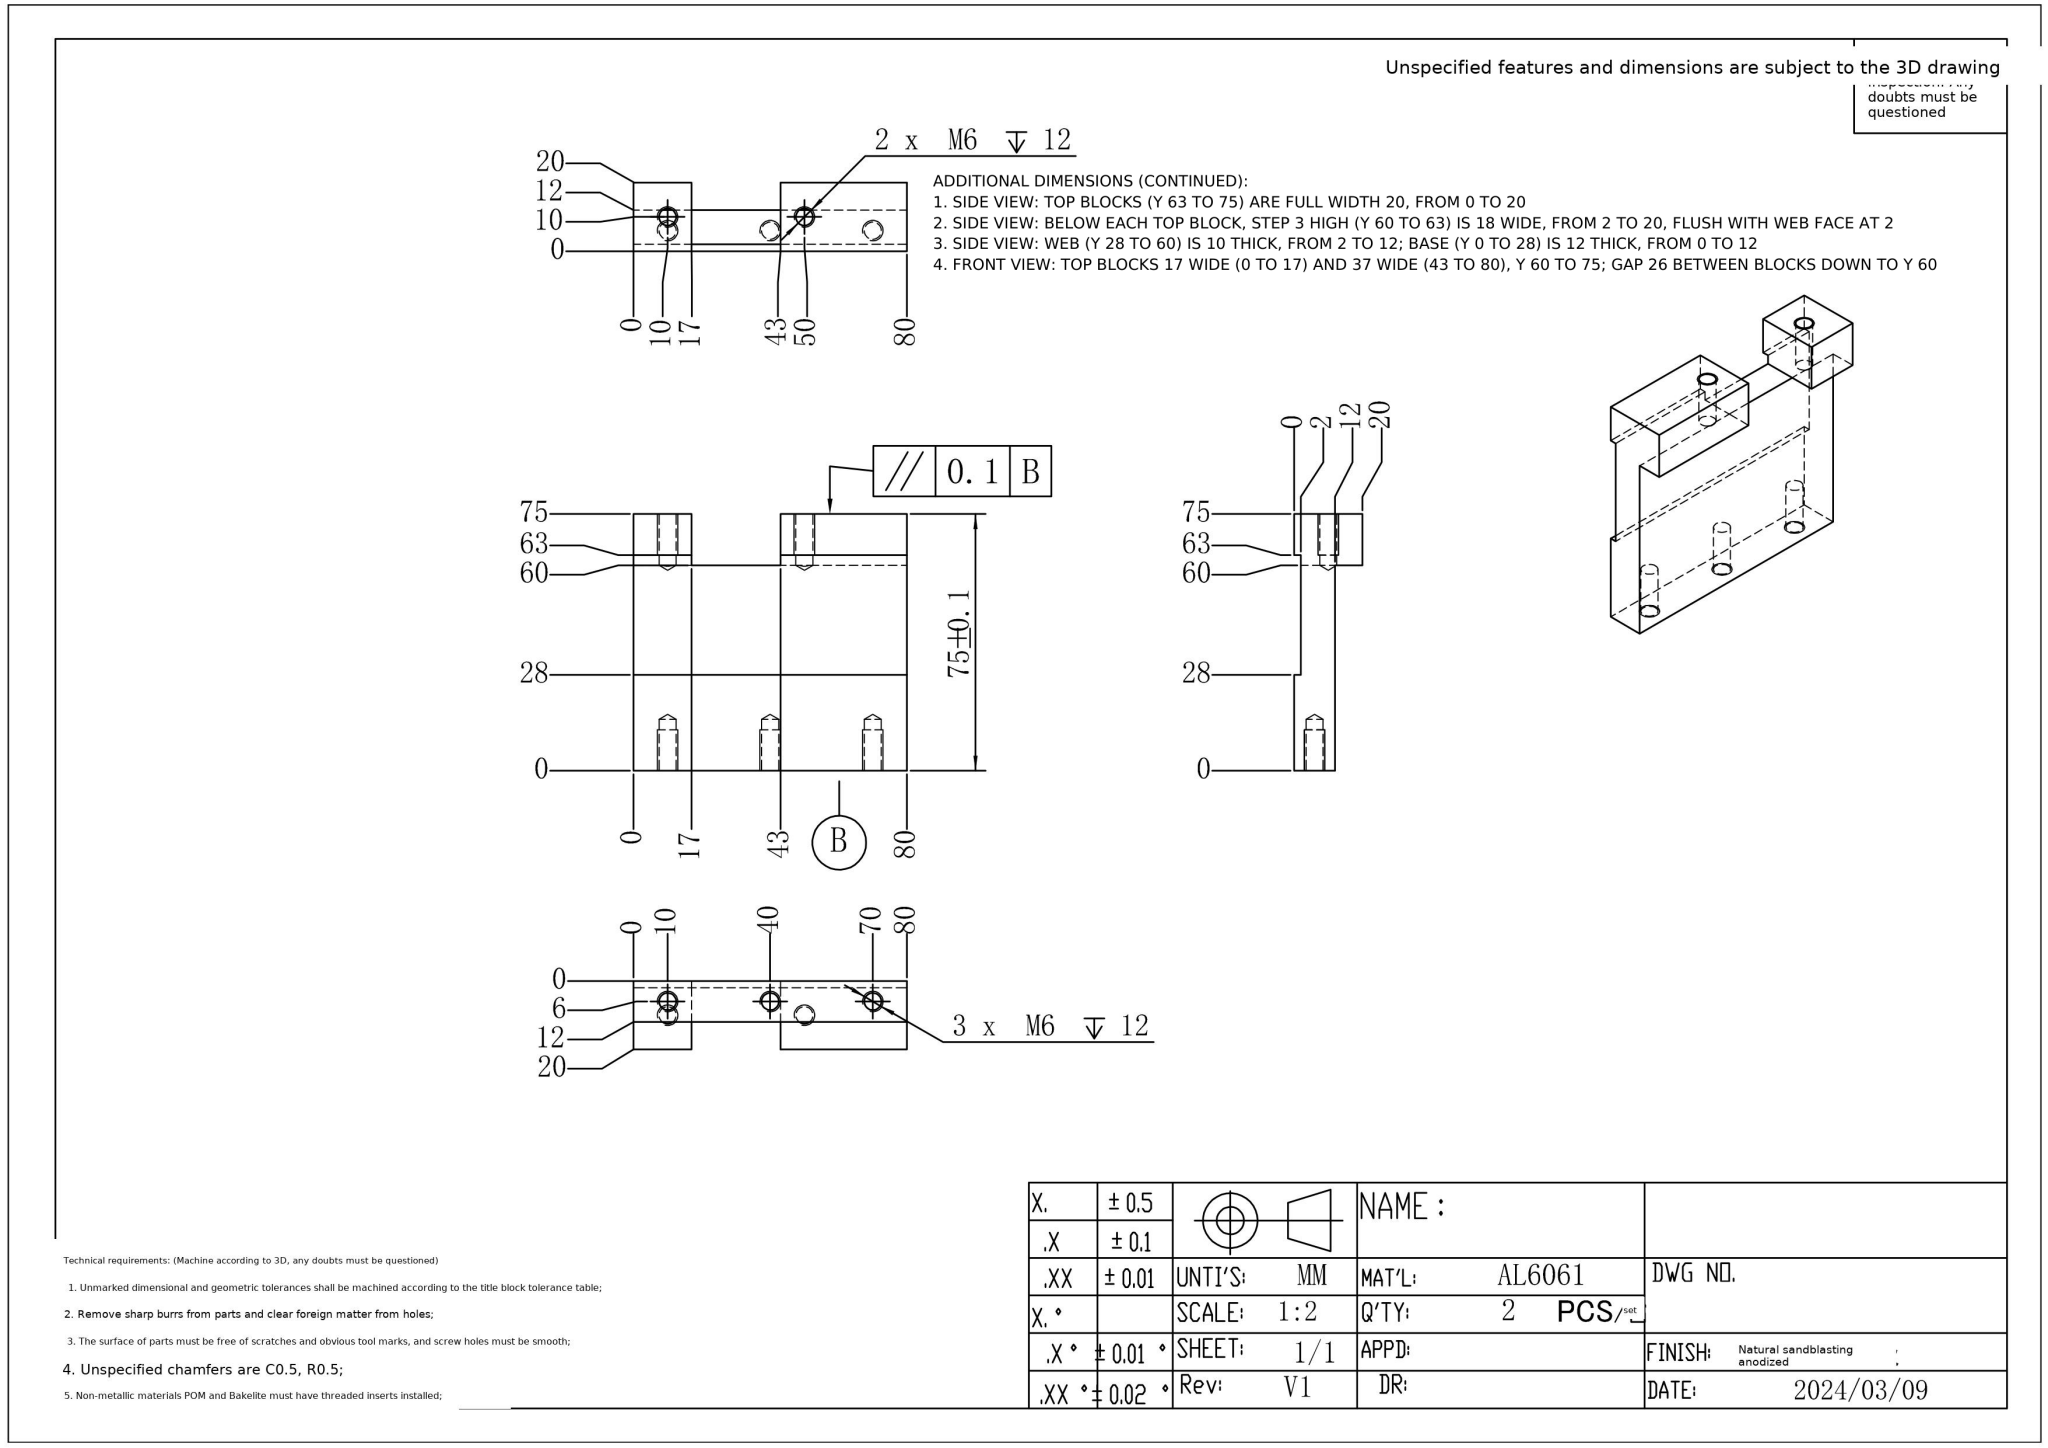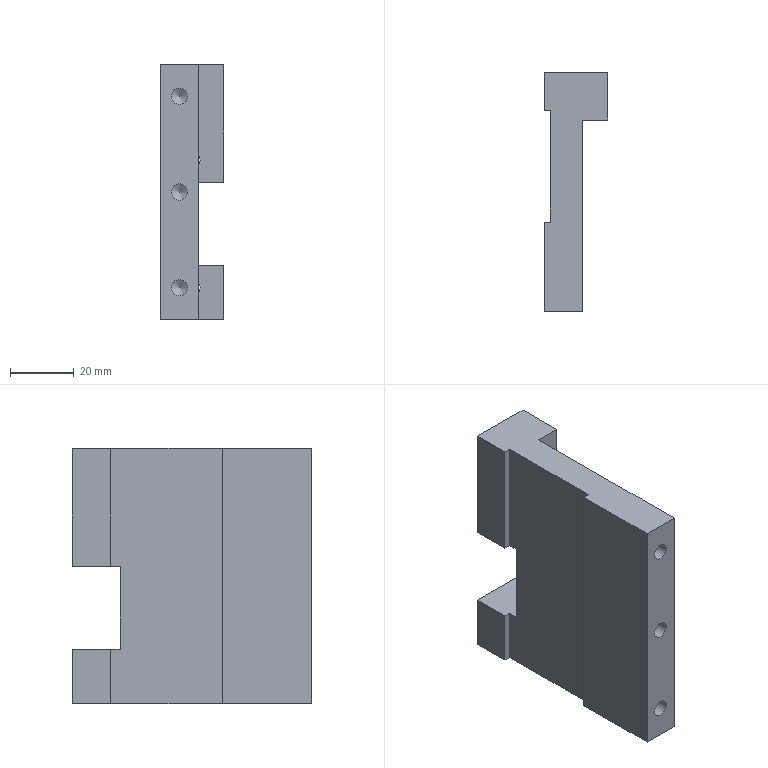Part | NX | mm | 1 solid | 30 faces | box 20 x 75 x 80 mm | volume 66772 mm3 | plane 20 | cone 5 | cylinder 5 | commonest cylinder face diameters 5.1 x5
STEP:
#1=CARTESIAN_POINT('',(0.,0.,0.));
#2=DIRECTION('',(0.,0.,1.));
#3=DIRECTION('',(1.,0.,0.));
#4=AXIS2_PLACEMENT_3D('',#1,#2,#3);
#5=(LENGTH_UNIT()NAMED_UNIT(*)SI_UNIT(.MILLI.,.METRE.));
#6=UNCERTAINTY_MEASURE_WITH_UNIT(LENGTH_MEASURE(0.0508),#5,'','');
#7=(NAMED_UNIT(*)PLANE_ANGLE_UNIT()SI_UNIT($,.RADIAN.));
#8=PLANE_ANGLE_MEASURE_WITH_UNIT(PLANE_ANGLE_MEASURE(0.01745),#7);
#9=DIMENSIONAL_EXPONENTS(0.,0.,0.,0.,0.,0.,0.);
#10=(CONVERSION_BASED_UNIT('',#8)NAMED_UNIT(#9)PLANE_ANGLE_UNIT());
#11=(NAMED_UNIT(*)SI_UNIT($,.STERADIAN.)SOLID_ANGLE_UNIT());
#12=(GEOMETRIC_REPRESENTATION_CONTEXT(3)GLOBAL_UNCERTAINTY_ASSIGNED_CONTEXT((#6))GLOBAL_UNIT_ASSIGNED_CONTEXT((#5,#10,#11))REPRESENTATION_CONTEXT('',''));
#13=SHAPE_REPRESENTATION('',(#4),#12);
#14=CARTESIAN_POINT('',(2.,60.,-63.));
#15=VERTEX_POINT('',#14);
#16=CARTESIAN_POINT('',(2.,60.,-37.));
#17=VERTEX_POINT('',#16);
#18=CARTESIAN_POINT('',(2.,60.,-80.));
#19=DIRECTION('',(0.,0.,1.));
#20=VECTOR('',#19,1.);
#21=LINE('',#18,#20);
#22=EDGE_CURVE('',#15,#17,#21,.T.);
#23=ORIENTED_EDGE('',*,*,#22,.T.);
#24=CARTESIAN_POINT('',(12.,60.,-37.));
#25=VERTEX_POINT('',#24);
#26=CARTESIAN_POINT('',(12.,60.,-37.));
#27=DIRECTION('',(-1.,0.,0.));
#28=VECTOR('',#27,1.);
#29=LINE('',#26,#28);
#30=EDGE_CURVE('',#25,#17,#29,.T.);
#31=ORIENTED_EDGE('',*,*,#30,.F.);
#32=CARTESIAN_POINT('',(12.,60.,-63.));
#33=VERTEX_POINT('',#32);
#34=CARTESIAN_POINT('',(12.,60.,-80.));
#35=DIRECTION('',(0.,0.,1.));
#36=VECTOR('',#35,1.);
#37=LINE('',#34,#36);
#38=EDGE_CURVE('',#33,#25,#37,.T.);
#39=ORIENTED_EDGE('',*,*,#38,.F.);
#40=CARTESIAN_POINT('',(2.,60.,-63.));
#41=DIRECTION('',(1.,0.,0.));
#42=VECTOR('',#41,1.);
#43=LINE('',#40,#42);
#44=EDGE_CURVE('',#15,#33,#43,.T.);
#45=ORIENTED_EDGE('',*,*,#44,.F.);
#46=EDGE_LOOP('',(#23,#31,#39,#45));
#47=FACE_OUTER_BOUND('',#46,.T.);
#48=CARTESIAN_POINT('',(12.,60.,-80.));
#49=DIRECTION('',(0.,1.,0.));
#50=DIRECTION('',(0.,0.,1.));
#51=AXIS2_PLACEMENT_3D('',#48,#49,#50);
#52=PLANE('',#51);
#53=ADVANCED_FACE('',(#47),#52,.T.);
#54=CARTESIAN_POINT('',(0.,28.,0.));
#55=VERTEX_POINT('',#54);
#56=CARTESIAN_POINT('',(0.,0.,0.));
#57=VERTEX_POINT('',#56);
#58=CARTESIAN_POINT('',(0.,28.,0.));
#59=DIRECTION('',(-0.,-1.,0.));
#60=VECTOR('',#59,1.);
#61=LINE('',#58,#60);
#62=EDGE_CURVE('',#55,#57,#61,.T.);
#63=ORIENTED_EDGE('',*,*,#62,.F.);
#64=CARTESIAN_POINT('',(0.,28.,-80.));
#65=VERTEX_POINT('',#64);
#66=CARTESIAN_POINT('',(0.,28.,-80.));
#67=DIRECTION('',(0.,0.,1.));
#68=VECTOR('',#67,1.);
#69=LINE('',#66,#68);
#70=EDGE_CURVE('',#65,#55,#69,.T.);
#71=ORIENTED_EDGE('',*,*,#70,.F.);
#72=CARTESIAN_POINT('',(0.,0.,-80.));
#73=VERTEX_POINT('',#72);
#74=CARTESIAN_POINT('',(0.,28.,-80.));
#75=DIRECTION('',(-0.,-1.,0.));
#76=VECTOR('',#75,1.);
#77=LINE('',#74,#76);
#78=EDGE_CURVE('',#65,#73,#77,.T.);
#79=ORIENTED_EDGE('',*,*,#78,.T.);
#80=CARTESIAN_POINT('',(0.,0.,-80.));
#81=DIRECTION('',(0.,0.,1.));
#82=VECTOR('',#81,1.);
#83=LINE('',#80,#82);
#84=EDGE_CURVE('',#73,#57,#83,.T.);
#85=ORIENTED_EDGE('',*,*,#84,.T.);
#86=EDGE_LOOP('',(#63,#71,#79,#85));
#87=FACE_OUTER_BOUND('',#86,.T.);
#88=CARTESIAN_POINT('',(0.,28.,-80.));
#89=DIRECTION('',(-1.,0.,0.));
#90=DIRECTION('',(-0.,-1.,0.));
#91=AXIS2_PLACEMENT_3D('',#88,#89,#90);
#92=PLANE('',#91);
#93=ADVANCED_FACE('',(#87),#92,.T.);
#94=CARTESIAN_POINT('',(3.45,0.,-40.));
#95=VERTEX_POINT('',#94);
#96=CARTESIAN_POINT('',(6.,0.,-40.));
#97=DIRECTION('',(0.,1.,0.));
#98=DIRECTION('',(-1.,0.,0.));
#99=AXIS2_PLACEMENT_3D('',#96,#97,#98);
#100=CIRCLE('',#99,2.55);
#101=EDGE_CURVE('',#95,#95,#100,.T.);
#102=ORIENTED_EDGE('',*,*,#101,.T.);
#103=EDGE_LOOP('',(#102));
#104=FACE_BOUND('',#103,.T.);
#105=CARTESIAN_POINT('',(3.45,0.,-10.));
#106=VERTEX_POINT('',#105);
#107=CARTESIAN_POINT('',(6.,0.,-10.));
#108=DIRECTION('',(0.,1.,0.));
#109=DIRECTION('',(-1.,0.,0.));
#110=AXIS2_PLACEMENT_3D('',#107,#108,#109);
#111=CIRCLE('',#110,2.55);
#112=EDGE_CURVE('',#106,#106,#111,.T.);
#113=ORIENTED_EDGE('',*,*,#112,.T.);
#114=EDGE_LOOP('',(#113));
#115=FACE_BOUND('',#114,.T.);
#116=CARTESIAN_POINT('',(3.45,0.,-70.));
#117=VERTEX_POINT('',#116);
#118=CARTESIAN_POINT('',(6.,0.,-70.));
#119=DIRECTION('',(0.,1.,0.));
#120=DIRECTION('',(-1.,0.,0.));
#121=AXIS2_PLACEMENT_3D('',#118,#119,#120);
#122=CIRCLE('',#121,2.55);
#123=EDGE_CURVE('',#117,#117,#122,.T.);
#124=ORIENTED_EDGE('',*,*,#123,.T.);
#125=EDGE_LOOP('',(#124));
#126=FACE_BOUND('',#125,.T.);
#127=CARTESIAN_POINT('',(12.,0.,0.));
#128=VERTEX_POINT('',#127);
#129=CARTESIAN_POINT('',(0.,0.,0.));
#130=DIRECTION('',(1.,-0.,0.));
#131=VECTOR('',#130,1.);
#132=LINE('',#129,#131);
#133=EDGE_CURVE('',#57,#128,#132,.T.);
#134=ORIENTED_EDGE('',*,*,#133,.F.);
#135=ORIENTED_EDGE('',*,*,#84,.F.);
#136=CARTESIAN_POINT('',(12.,0.,-80.));
#137=VERTEX_POINT('',#136);
#138=CARTESIAN_POINT('',(0.,0.,-80.));
#139=DIRECTION('',(1.,-0.,0.));
#140=VECTOR('',#139,1.);
#141=LINE('',#138,#140);
#142=EDGE_CURVE('',#73,#137,#141,.T.);
#143=ORIENTED_EDGE('',*,*,#142,.T.);
#144=CARTESIAN_POINT('',(12.,0.,-80.));
#145=DIRECTION('',(0.,0.,1.));
#146=VECTOR('',#145,1.);
#147=LINE('',#144,#146);
#148=EDGE_CURVE('',#137,#128,#147,.T.);
#149=ORIENTED_EDGE('',*,*,#148,.T.);
#150=EDGE_LOOP('',(#134,#135,#143,#149));
#151=FACE_BOUND('',#150,.T.);
#152=CARTESIAN_POINT('',(0.,0.,-80.));
#153=DIRECTION('',(-0.,-1.,0.));
#154=DIRECTION('',(1.,-0.,0.));
#155=AXIS2_PLACEMENT_3D('',#152,#153,#154);
#156=PLANE('',#155);
#157=ADVANCED_FACE('',(#104,#115,#126,#151),#156,.T.);
#158=CARTESIAN_POINT('',(12.,60.,-68.418));
#159=VERTEX_POINT('',#158);
#160=CARTESIAN_POINT('',(12.,60.,-71.582));
#161=VERTEX_POINT('',#160);
#162=CARTESIAN_POINT('',(12.,60.,-68.418));
#163=CARTESIAN_POINT('',(12.,59.81,-68.928));
#164=CARTESIAN_POINT('',(12.,59.669,-69.462));
#165=CARTESIAN_POINT('',(12.,59.67,-70.546));
#166=CARTESIAN_POINT('',(12.,59.811,-71.075));
#167=CARTESIAN_POINT('',(12.,60.,-71.582));
#168=B_SPLINE_CURVE_WITH_KNOTS('',3,(#162,#163,#164,#165,#166,#167),.UNSPECIFIED.,.F.,.F.,(4,2,4),(0.,0.5,1.),.UNSPECIFIED.);
#169=EDGE_CURVE('',#159,#161,#168,.T.);
#170=ORIENTED_EDGE('',*,*,#169,.F.);
#171=CARTESIAN_POINT('',(12.,60.,-80.));
#172=DIRECTION('',(0.,0.,1.));
#173=VECTOR('',#172,1.);
#174=LINE('',#171,#173);
#175=EDGE_CURVE('',#159,#33,#174,.T.);
#176=ORIENTED_EDGE('',*,*,#175,.T.);
#177=ORIENTED_EDGE('',*,*,#38,.T.);
#178=CARTESIAN_POINT('',(12.,60.,-31.582));
#179=VERTEX_POINT('',#178);
#180=CARTESIAN_POINT('',(12.,60.,-80.));
#181=DIRECTION('',(0.,0.,1.));
#182=VECTOR('',#181,1.);
#183=LINE('',#180,#182);
#184=EDGE_CURVE('',#25,#179,#183,.T.);
#185=ORIENTED_EDGE('',*,*,#184,.T.);
#186=CARTESIAN_POINT('',(12.,60.,-28.418));
#187=VERTEX_POINT('',#186);
#188=CARTESIAN_POINT('',(12.,60.,-28.418));
#189=CARTESIAN_POINT('',(12.,59.81,-28.928));
#190=CARTESIAN_POINT('',(12.,59.669,-29.462));
#191=CARTESIAN_POINT('',(12.,59.67,-30.546));
#192=CARTESIAN_POINT('',(12.,59.811,-31.075));
#193=CARTESIAN_POINT('',(12.,60.,-31.582));
#194=B_SPLINE_CURVE_WITH_KNOTS('',3,(#188,#189,#190,#191,#192,#193),.UNSPECIFIED.,.F.,.F.,(4,2,4),(0.,0.5,1.),.UNSPECIFIED.);
#195=EDGE_CURVE('',#187,#179,#194,.T.);
#196=ORIENTED_EDGE('',*,*,#195,.F.);
#197=CARTESIAN_POINT('',(12.,60.,0.));
#198=VERTEX_POINT('',#197);
#199=CARTESIAN_POINT('',(12.,60.,-80.));
#200=DIRECTION('',(0.,0.,1.));
#201=VECTOR('',#200,1.);
#202=LINE('',#199,#201);
#203=EDGE_CURVE('',#187,#198,#202,.T.);
#204=ORIENTED_EDGE('',*,*,#203,.T.);
#205=CARTESIAN_POINT('',(12.,0.,0.));
#206=DIRECTION('',(-0.,1.,0.));
#207=VECTOR('',#206,1.);
#208=LINE('',#205,#207);
#209=EDGE_CURVE('',#128,#198,#208,.T.);
#210=ORIENTED_EDGE('',*,*,#209,.F.);
#211=ORIENTED_EDGE('',*,*,#148,.F.);
#212=CARTESIAN_POINT('',(12.,60.,-80.));
#213=VERTEX_POINT('',#212);
#214=CARTESIAN_POINT('',(12.,0.,-80.));
#215=DIRECTION('',(-0.,1.,0.));
#216=VECTOR('',#215,1.);
#217=LINE('',#214,#216);
#218=EDGE_CURVE('',#137,#213,#217,.T.);
#219=ORIENTED_EDGE('',*,*,#218,.T.);
#220=CARTESIAN_POINT('',(12.,60.,-80.));
#221=DIRECTION('',(0.,0.,1.));
#222=VECTOR('',#221,1.);
#223=LINE('',#220,#222);
#224=EDGE_CURVE('',#213,#161,#223,.T.);
#225=ORIENTED_EDGE('',*,*,#224,.T.);
#226=EDGE_LOOP('',(#170,#176,#177,#185,#196,#204,#210,#211,#219,#225));
#227=FACE_OUTER_BOUND('',#226,.T.);
#228=CARTESIAN_POINT('',(12.,0.,-80.));
#229=DIRECTION('',(1.,0.,0.));
#230=DIRECTION('',(-0.,1.,0.));
#231=AXIS2_PLACEMENT_3D('',#228,#229,#230);
#232=PLANE('',#231);
#233=ADVANCED_FACE('',(#227),#232,.T.);
#234=CARTESIAN_POINT('',(2.,63.,0.));
#235=VERTEX_POINT('',#234);
#236=CARTESIAN_POINT('',(2.,28.,0.));
#237=VERTEX_POINT('',#236);
#238=CARTESIAN_POINT('',(2.,60.,0.));
#239=DIRECTION('',(0.,-1.,0.));
#240=VECTOR('',#239,1.);
#241=LINE('',#238,#240);
#242=EDGE_CURVE('',#235,#237,#241,.T.);
#243=ORIENTED_EDGE('',*,*,#242,.F.);
#244=CARTESIAN_POINT('',(2.,63.,-37.));
#245=VERTEX_POINT('',#244);
#246=CARTESIAN_POINT('',(2.,63.,0.));
#247=DIRECTION('',(0.,0.,-1.));
#248=VECTOR('',#247,1.);
#249=LINE('',#246,#248);
#250=EDGE_CURVE('',#235,#245,#249,.T.);
#251=ORIENTED_EDGE('',*,*,#250,.T.);
#252=CARTESIAN_POINT('',(2.,63.,-37.));
#253=DIRECTION('',(0.,1.,0.));
#254=VECTOR('',#253,1.);
#255=LINE('',#252,#254);
#256=EDGE_CURVE('',#17,#245,#255,.T.);
#257=ORIENTED_EDGE('',*,*,#256,.F.);
#258=ORIENTED_EDGE('',*,*,#22,.F.);
#259=CARTESIAN_POINT('',(2.,63.,-63.));
#260=VERTEX_POINT('',#259);
#261=CARTESIAN_POINT('',(2.,63.,-63.));
#262=DIRECTION('',(0.,-1.,0.));
#263=VECTOR('',#262,1.);
#264=LINE('',#261,#263);
#265=EDGE_CURVE('',#260,#15,#264,.T.);
#266=ORIENTED_EDGE('',*,*,#265,.F.);
#267=CARTESIAN_POINT('',(2.,63.,-80.));
#268=VERTEX_POINT('',#267);
#269=CARTESIAN_POINT('',(2.,63.,-80.));
#270=DIRECTION('',(0.,0.,1.));
#271=VECTOR('',#270,1.);
#272=LINE('',#269,#271);
#273=EDGE_CURVE('',#268,#260,#272,.T.);
#274=ORIENTED_EDGE('',*,*,#273,.F.);
#275=CARTESIAN_POINT('',(2.,28.,-80.));
#276=VERTEX_POINT('',#275);
#277=CARTESIAN_POINT('',(2.,60.,-80.));
#278=DIRECTION('',(0.,-1.,0.));
#279=VECTOR('',#278,1.);
#280=LINE('',#277,#279);
#281=EDGE_CURVE('',#268,#276,#280,.T.);
#282=ORIENTED_EDGE('',*,*,#281,.T.);
#283=CARTESIAN_POINT('',(2.,28.,-80.));
#284=DIRECTION('',(0.,0.,1.));
#285=VECTOR('',#284,1.);
#286=LINE('',#283,#285);
#287=EDGE_CURVE('',#276,#237,#286,.T.);
#288=ORIENTED_EDGE('',*,*,#287,.T.);
#289=EDGE_LOOP('',(#243,#251,#257,#258,#266,#274,#282,#288));
#290=FACE_OUTER_BOUND('',#289,.T.);
#291=CARTESIAN_POINT('',(2.,60.,-80.));
#292=DIRECTION('',(-1.,-0.,0.));
#293=DIRECTION('',(0.,-1.,0.));
#294=AXIS2_PLACEMENT_3D('',#291,#292,#293);
#295=PLANE('',#294);
#296=ADVANCED_FACE('',(#290),#295,.T.);
#297=CARTESIAN_POINT('',(2.,28.,0.));
#298=DIRECTION('',(-1.,0.,0.));
#299=VECTOR('',#298,1.);
#300=LINE('',#297,#299);
#301=EDGE_CURVE('',#237,#55,#300,.T.);
#302=ORIENTED_EDGE('',*,*,#301,.F.);
#303=ORIENTED_EDGE('',*,*,#287,.F.);
#304=CARTESIAN_POINT('',(2.,28.,-80.));
#305=DIRECTION('',(-1.,0.,0.));
#306=VECTOR('',#305,1.);
#307=LINE('',#304,#306);
#308=EDGE_CURVE('',#276,#65,#307,.T.);
#309=ORIENTED_EDGE('',*,*,#308,.T.);
#310=ORIENTED_EDGE('',*,*,#70,.T.);
#311=EDGE_LOOP('',(#302,#303,#309,#310));
#312=FACE_OUTER_BOUND('',#311,.T.);
#313=CARTESIAN_POINT('',(2.,28.,-80.));
#314=DIRECTION('',(0.,1.,0.));
#315=DIRECTION('',(0.,0.,1.));
#316=AXIS2_PLACEMENT_3D('',#313,#314,#315);
#317=PLANE('',#316);
#318=ADVANCED_FACE('',(#312),#317,.T.);
#319=ORIENTED_EDGE('',*,*,#78,.F.);
#320=ORIENTED_EDGE('',*,*,#308,.F.);
#321=ORIENTED_EDGE('',*,*,#281,.F.);
#322=CARTESIAN_POINT('',(-0.,63.,-80.));
#323=VERTEX_POINT('',#322);
#324=CARTESIAN_POINT('',(-0.,63.,-80.));
#325=DIRECTION('',(1.,0.,0.));
#326=VECTOR('',#325,1.);
#327=LINE('',#324,#326);
#328=EDGE_CURVE('',#323,#268,#327,.T.);
#329=ORIENTED_EDGE('',*,*,#328,.F.);
#330=CARTESIAN_POINT('',(-0.,75.,-80.));
#331=VERTEX_POINT('',#330);
#332=CARTESIAN_POINT('',(-0.,75.,-80.));
#333=DIRECTION('',(0.,-1.,0.));
#334=VECTOR('',#333,1.);
#335=LINE('',#332,#334);
#336=EDGE_CURVE('',#331,#323,#335,.T.);
#337=ORIENTED_EDGE('',*,*,#336,.F.);
#338=CARTESIAN_POINT('',(20.,75.,-80.));
#339=VERTEX_POINT('',#338);
#340=CARTESIAN_POINT('',(20.,75.,-80.));
#341=DIRECTION('',(-1.,0.,0.));
#342=VECTOR('',#341,1.);
#343=LINE('',#340,#342);
#344=EDGE_CURVE('',#339,#331,#343,.T.);
#345=ORIENTED_EDGE('',*,*,#344,.F.);
#346=CARTESIAN_POINT('',(20.,60.,-80.));
#347=VERTEX_POINT('',#346);
#348=CARTESIAN_POINT('',(20.,60.,-80.));
#349=DIRECTION('',(0.,1.,0.));
#350=VECTOR('',#349,1.);
#351=LINE('',#348,#350);
#352=EDGE_CURVE('',#347,#339,#351,.T.);
#353=ORIENTED_EDGE('',*,*,#352,.F.);
#354=CARTESIAN_POINT('',(2.,60.,-80.));
#355=DIRECTION('',(1.,0.,0.));
#356=VECTOR('',#355,1.);
#357=LINE('',#354,#356);
#358=EDGE_CURVE('',#213,#347,#357,.T.);
#359=ORIENTED_EDGE('',*,*,#358,.F.);
#360=ORIENTED_EDGE('',*,*,#218,.F.);
#361=ORIENTED_EDGE('',*,*,#142,.F.);
#362=EDGE_LOOP('',(#319,#320,#321,#329,#337,#345,#353,#359,#360,#361));
#363=FACE_OUTER_BOUND('',#362,.T.);
#364=CARTESIAN_POINT('',(0.,0.,-80.));
#365=DIRECTION('',(0.,0.,1.));
#366=DIRECTION('',(1.,0.,0.));
#367=AXIS2_PLACEMENT_3D('',#364,#365,#366);
#368=PLANE('',#367);
#369=ADVANCED_FACE('',(#363),#368,.F.);
#370=ORIENTED_EDGE('',*,*,#62,.T.);
#371=ORIENTED_EDGE('',*,*,#133,.T.);
#372=ORIENTED_EDGE('',*,*,#209,.T.);
#373=CARTESIAN_POINT('',(20.,60.,0.));
#374=VERTEX_POINT('',#373);
#375=CARTESIAN_POINT('',(2.,60.,0.));
#376=DIRECTION('',(1.,0.,0.));
#377=VECTOR('',#376,1.);
#378=LINE('',#375,#377);
#379=EDGE_CURVE('',#198,#374,#378,.T.);
#380=ORIENTED_EDGE('',*,*,#379,.T.);
#381=CARTESIAN_POINT('',(20.,75.,0.));
#382=VERTEX_POINT('',#381);
#383=CARTESIAN_POINT('',(20.,60.,0.));
#384=DIRECTION('',(0.,1.,0.));
#385=VECTOR('',#384,1.);
#386=LINE('',#383,#385);
#387=EDGE_CURVE('',#374,#382,#386,.T.);
#388=ORIENTED_EDGE('',*,*,#387,.T.);
#389=CARTESIAN_POINT('',(-0.,75.,0.));
#390=VERTEX_POINT('',#389);
#391=CARTESIAN_POINT('',(20.,75.,0.));
#392=DIRECTION('',(-1.,0.,0.));
#393=VECTOR('',#392,1.);
#394=LINE('',#391,#393);
#395=EDGE_CURVE('',#382,#390,#394,.T.);
#396=ORIENTED_EDGE('',*,*,#395,.T.);
#397=CARTESIAN_POINT('',(-0.,63.,0.));
#398=VERTEX_POINT('',#397);
#399=CARTESIAN_POINT('',(-0.,75.,0.));
#400=DIRECTION('',(0.,-1.,0.));
#401=VECTOR('',#400,1.);
#402=LINE('',#399,#401);
#403=EDGE_CURVE('',#390,#398,#402,.T.);
#404=ORIENTED_EDGE('',*,*,#403,.T.);
#405=CARTESIAN_POINT('',(-0.,63.,0.));
#406=DIRECTION('',(1.,0.,0.));
#407=VECTOR('',#406,1.);
#408=LINE('',#405,#407);
#409=EDGE_CURVE('',#398,#235,#408,.T.);
#410=ORIENTED_EDGE('',*,*,#409,.T.);
#411=ORIENTED_EDGE('',*,*,#242,.T.);
#412=ORIENTED_EDGE('',*,*,#301,.T.);
#413=EDGE_LOOP('',(#370,#371,#372,#380,#388,#396,#404,#410,#411,#412));
#414=FACE_OUTER_BOUND('',#413,.T.);
#415=CARTESIAN_POINT('',(0.,0.,0.));
#416=DIRECTION('',(0.,0.,1.));
#417=DIRECTION('',(1.,0.,0.));
#418=AXIS2_PLACEMENT_3D('',#415,#416,#417);
#419=PLANE('',#418);
#420=ADVANCED_FACE('',(#414),#419,.T.);
#421=CARTESIAN_POINT('',(10.,60.,-70.));
#422=DIRECTION('',(0.,-1.,0.));
#423=DIRECTION('',(0.,0.,-1.));
#424=AXIS2_PLACEMENT_3D('',#421,#422,#423);
#425=CIRCLE('',#424,2.55);
#426=EDGE_CURVE('',#161,#159,#425,.T.);
#427=ORIENTED_EDGE('',*,*,#426,.F.);
#428=ORIENTED_EDGE('',*,*,#224,.F.);
#429=ORIENTED_EDGE('',*,*,#358,.T.);
#430=CARTESIAN_POINT('',(20.,60.,-63.));
#431=VERTEX_POINT('',#430);
#432=CARTESIAN_POINT('',(20.,60.,-80.));
#433=DIRECTION('',(0.,0.,1.));
#434=VECTOR('',#433,1.);
#435=LINE('',#432,#434);
#436=EDGE_CURVE('',#347,#431,#435,.T.);
#437=ORIENTED_EDGE('',*,*,#436,.T.);
#438=CARTESIAN_POINT('',(2.,60.,-63.));
#439=DIRECTION('',(1.,0.,0.));
#440=VECTOR('',#439,1.);
#441=LINE('',#438,#440);
#442=EDGE_CURVE('',#33,#431,#441,.T.);
#443=ORIENTED_EDGE('',*,*,#442,.F.);
#444=ORIENTED_EDGE('',*,*,#175,.F.);
#445=EDGE_LOOP('',(#427,#428,#429,#437,#443,#444));
#446=FACE_OUTER_BOUND('',#445,.T.);
#447=CARTESIAN_POINT('',(2.,60.,-80.));
#448=DIRECTION('',(0.,-1.,0.));
#449=DIRECTION('',(0.,0.,-1.));
#450=AXIS2_PLACEMENT_3D('',#447,#448,#449);
#451=PLANE('',#450);
#452=ADVANCED_FACE('',(#446),#451,.T.);
#453=CARTESIAN_POINT('',(-0.,75.,-63.));
#454=VERTEX_POINT('',#453);
#455=CARTESIAN_POINT('',(-0.,63.,-63.));
#456=VERTEX_POINT('',#455);
#457=CARTESIAN_POINT('',(-0.,75.,-63.));
#458=DIRECTION('',(0.,-1.,0.));
#459=VECTOR('',#458,1.);
#460=LINE('',#457,#459);
#461=EDGE_CURVE('',#454,#456,#460,.T.);
#462=ORIENTED_EDGE('',*,*,#461,.F.);
#463=CARTESIAN_POINT('',(-0.,75.,-80.));
#464=DIRECTION('',(0.,0.,1.));
#465=VECTOR('',#464,1.);
#466=LINE('',#463,#465);
#467=EDGE_CURVE('',#331,#454,#466,.T.);
#468=ORIENTED_EDGE('',*,*,#467,.F.);
#469=ORIENTED_EDGE('',*,*,#336,.T.);
#470=CARTESIAN_POINT('',(-0.,63.,-80.));
#471=DIRECTION('',(0.,0.,1.));
#472=VECTOR('',#471,1.);
#473=LINE('',#470,#472);
#474=EDGE_CURVE('',#323,#456,#473,.T.);
#475=ORIENTED_EDGE('',*,*,#474,.T.);
#476=EDGE_LOOP('',(#462,#468,#469,#475));
#477=FACE_OUTER_BOUND('',#476,.T.);
#478=CARTESIAN_POINT('',(-0.,75.,-80.));
#479=DIRECTION('',(-1.,-0.,0.));
#480=DIRECTION('',(0.,-1.,0.));
#481=AXIS2_PLACEMENT_3D('',#478,#479,#480);
#482=PLANE('',#481);
#483=ADVANCED_FACE('',(#477),#482,.T.);
#484=CARTESIAN_POINT('',(-0.,63.,-63.));
#485=DIRECTION('',(1.,0.,0.));
#486=VECTOR('',#485,1.);
#487=LINE('',#484,#486);
#488=EDGE_CURVE('',#456,#260,#487,.T.);
#489=ORIENTED_EDGE('',*,*,#488,.F.);
#490=ORIENTED_EDGE('',*,*,#474,.F.);
#491=ORIENTED_EDGE('',*,*,#328,.T.);
#492=ORIENTED_EDGE('',*,*,#273,.T.);
#493=EDGE_LOOP('',(#489,#490,#491,#492));
#494=FACE_OUTER_BOUND('',#493,.T.);
#495=CARTESIAN_POINT('',(-0.,63.,-80.));
#496=DIRECTION('',(0.,-1.,0.));
#497=DIRECTION('',(0.,0.,-1.));
#498=AXIS2_PLACEMENT_3D('',#495,#496,#497);
#499=PLANE('',#498);
#500=ADVANCED_FACE('',(#494),#499,.T.);
#501=CARTESIAN_POINT('',(20.,75.,-63.));
#502=VERTEX_POINT('',#501);
#503=CARTESIAN_POINT('',(20.,60.,-63.));
#504=DIRECTION('',(0.,1.,0.));
#505=VECTOR('',#504,1.);
#506=LINE('',#503,#505);
#507=EDGE_CURVE('',#431,#502,#506,.T.);
#508=ORIENTED_EDGE('',*,*,#507,.F.);
#509=ORIENTED_EDGE('',*,*,#436,.F.);
#510=ORIENTED_EDGE('',*,*,#352,.T.);
#511=CARTESIAN_POINT('',(20.,75.,-80.));
#512=DIRECTION('',(0.,0.,1.));
#513=VECTOR('',#512,1.);
#514=LINE('',#511,#513);
#515=EDGE_CURVE('',#339,#502,#514,.T.);
#516=ORIENTED_EDGE('',*,*,#515,.T.);
#517=EDGE_LOOP('',(#508,#509,#510,#516));
#518=FACE_OUTER_BOUND('',#517,.T.);
#519=CARTESIAN_POINT('',(20.,60.,-80.));
#520=DIRECTION('',(1.,0.,0.));
#521=DIRECTION('',(0.,0.,-1.));
#522=AXIS2_PLACEMENT_3D('',#519,#520,#521);
#523=PLANE('',#522);
#524=ADVANCED_FACE('',(#518),#523,.T.);
#525=CARTESIAN_POINT('',(10.,75.,-72.55));
#526=VERTEX_POINT('',#525);
#527=CARTESIAN_POINT('',(10.,75.,-70.));
#528=DIRECTION('',(0.,-1.,0.));
#529=DIRECTION('',(0.,0.,-1.));
#530=AXIS2_PLACEMENT_3D('',#527,#528,#529);
#531=CIRCLE('',#530,2.55);
#532=EDGE_CURVE('',#526,#526,#531,.T.);
#533=ORIENTED_EDGE('',*,*,#532,.T.);
#534=EDGE_LOOP('',(#533));
#535=FACE_BOUND('',#534,.T.);
#536=CARTESIAN_POINT('',(20.,75.,-63.));
#537=DIRECTION('',(-1.,0.,0.));
#538=VECTOR('',#537,1.);
#539=LINE('',#536,#538);
#540=EDGE_CURVE('',#502,#454,#539,.T.);
#541=ORIENTED_EDGE('',*,*,#540,.F.);
#542=ORIENTED_EDGE('',*,*,#515,.F.);
#543=ORIENTED_EDGE('',*,*,#344,.T.);
#544=ORIENTED_EDGE('',*,*,#467,.T.);
#545=EDGE_LOOP('',(#541,#542,#543,#544));
#546=FACE_BOUND('',#545,.T.);
#547=CARTESIAN_POINT('',(20.,75.,-80.));
#548=DIRECTION('',(0.,1.,0.));
#549=DIRECTION('',(0.,0.,1.));
#550=AXIS2_PLACEMENT_3D('',#547,#548,#549);
#551=PLANE('',#550);
#552=ADVANCED_FACE('',(#535,#546),#551,.T.);
#553=ORIENTED_EDGE('',*,*,#461,.T.);
#554=ORIENTED_EDGE('',*,*,#488,.T.);
#555=ORIENTED_EDGE('',*,*,#265,.T.);
#556=ORIENTED_EDGE('',*,*,#44,.T.);
#557=ORIENTED_EDGE('',*,*,#442,.T.);
#558=ORIENTED_EDGE('',*,*,#507,.T.);
#559=ORIENTED_EDGE('',*,*,#540,.T.);
#560=EDGE_LOOP('',(#553,#554,#555,#556,#557,#558,#559));
#561=FACE_OUTER_BOUND('',#560,.T.);
#562=CARTESIAN_POINT('',(0.,0.,-63.));
#563=DIRECTION('',(0.,0.,1.));
#564=DIRECTION('',(1.,0.,0.));
#565=AXIS2_PLACEMENT_3D('',#562,#563,#564);
#566=PLANE('',#565);
#567=ADVANCED_FACE('',(#561),#566,.T.);
#568=CARTESIAN_POINT('',(-0.,75.,-37.));
#569=VERTEX_POINT('',#568);
#570=CARTESIAN_POINT('',(-0.,63.,-37.));
#571=VERTEX_POINT('',#570);
#572=CARTESIAN_POINT('',(-0.,75.,-37.));
#573=DIRECTION('',(0.,-1.,0.));
#574=VECTOR('',#573,1.);
#575=LINE('',#572,#574);
#576=EDGE_CURVE('',#569,#571,#575,.T.);
#577=ORIENTED_EDGE('',*,*,#576,.T.);
#578=CARTESIAN_POINT('',(-0.,63.,0.));
#579=DIRECTION('',(0.,0.,-1.));
#580=VECTOR('',#579,1.);
#581=LINE('',#578,#580);
#582=EDGE_CURVE('',#398,#571,#581,.T.);
#583=ORIENTED_EDGE('',*,*,#582,.F.);
#584=ORIENTED_EDGE('',*,*,#403,.F.);
#585=CARTESIAN_POINT('',(-0.,75.,0.));
#586=DIRECTION('',(0.,0.,-1.));
#587=VECTOR('',#586,1.);
#588=LINE('',#585,#587);
#589=EDGE_CURVE('',#390,#569,#588,.T.);
#590=ORIENTED_EDGE('',*,*,#589,.T.);
#591=EDGE_LOOP('',(#577,#583,#584,#590));
#592=FACE_OUTER_BOUND('',#591,.T.);
#593=CARTESIAN_POINT('',(-0.,75.,0.));
#594=DIRECTION('',(1.,0.,0.));
#595=DIRECTION('',(-0.,1.,0.));
#596=AXIS2_PLACEMENT_3D('',#593,#594,#595);
#597=PLANE('',#596);
#598=ADVANCED_FACE('',(#592),#597,.F.);
#599=CARTESIAN_POINT('',(-0.,63.,-37.));
#600=DIRECTION('',(1.,0.,0.));
#601=VECTOR('',#600,1.);
#602=LINE('',#599,#601);
#603=EDGE_CURVE('',#571,#245,#602,.T.);
#604=ORIENTED_EDGE('',*,*,#603,.T.);
#605=ORIENTED_EDGE('',*,*,#250,.F.);
#606=ORIENTED_EDGE('',*,*,#409,.F.);
#607=ORIENTED_EDGE('',*,*,#582,.T.);
#608=EDGE_LOOP('',(#604,#605,#606,#607));
#609=FACE_OUTER_BOUND('',#608,.T.);
#610=CARTESIAN_POINT('',(-0.,63.,0.));
#611=DIRECTION('',(0.,1.,0.));
#612=DIRECTION('',(0.,0.,1.));
#613=AXIS2_PLACEMENT_3D('',#610,#611,#612);
#614=PLANE('',#613);
#615=ADVANCED_FACE('',(#609),#614,.F.);
#616=ORIENTED_EDGE('',*,*,#203,.F.);
#617=CARTESIAN_POINT('',(10.,60.,-30.));
#618=DIRECTION('',(0.,-1.,0.));
#619=DIRECTION('',(0.,0.,-1.));
#620=AXIS2_PLACEMENT_3D('',#617,#618,#619);
#621=CIRCLE('',#620,2.55);
#622=EDGE_CURVE('',#179,#187,#621,.T.);
#623=ORIENTED_EDGE('',*,*,#622,.F.);
#624=ORIENTED_EDGE('',*,*,#184,.F.);
#625=CARTESIAN_POINT('',(20.,60.,-37.));
#626=VERTEX_POINT('',#625);
#627=CARTESIAN_POINT('',(12.,60.,-37.));
#628=DIRECTION('',(1.,0.,0.));
#629=VECTOR('',#628,1.);
#630=LINE('',#627,#629);
#631=EDGE_CURVE('',#25,#626,#630,.T.);
#632=ORIENTED_EDGE('',*,*,#631,.T.);
#633=CARTESIAN_POINT('',(20.,60.,0.));
#634=DIRECTION('',(0.,0.,-1.));
#635=VECTOR('',#634,1.);
#636=LINE('',#633,#635);
#637=EDGE_CURVE('',#374,#626,#636,.T.);
#638=ORIENTED_EDGE('',*,*,#637,.F.);
#639=ORIENTED_EDGE('',*,*,#379,.F.);
#640=EDGE_LOOP('',(#616,#623,#624,#632,#638,#639));
#641=FACE_OUTER_BOUND('',#640,.T.);
#642=CARTESIAN_POINT('',(12.,60.,0.));
#643=DIRECTION('',(0.,1.,0.));
#644=DIRECTION('',(0.,0.,1.));
#645=AXIS2_PLACEMENT_3D('',#642,#643,#644);
#646=PLANE('',#645);
#647=ADVANCED_FACE('',(#641),#646,.F.);
#648=CARTESIAN_POINT('',(20.,75.,-37.));
#649=VERTEX_POINT('',#648);
#650=CARTESIAN_POINT('',(20.,60.,-37.));
#651=DIRECTION('',(0.,1.,0.));
#652=VECTOR('',#651,1.);
#653=LINE('',#650,#652);
#654=EDGE_CURVE('',#626,#649,#653,.T.);
#655=ORIENTED_EDGE('',*,*,#654,.T.);
#656=CARTESIAN_POINT('',(20.,75.,0.));
#657=DIRECTION('',(0.,0.,-1.));
#658=VECTOR('',#657,1.);
#659=LINE('',#656,#658);
#660=EDGE_CURVE('',#382,#649,#659,.T.);
#661=ORIENTED_EDGE('',*,*,#660,.F.);
#662=ORIENTED_EDGE('',*,*,#387,.F.);
#663=ORIENTED_EDGE('',*,*,#637,.T.);
#664=EDGE_LOOP('',(#655,#661,#662,#663));
#665=FACE_OUTER_BOUND('',#664,.T.);
#666=CARTESIAN_POINT('',(20.,60.,0.));
#667=DIRECTION('',(-1.,0.,0.));
#668=DIRECTION('',(0.,0.,1.));
#669=AXIS2_PLACEMENT_3D('',#666,#667,#668);
#670=PLANE('',#669);
#671=ADVANCED_FACE('',(#665),#670,.F.);
#672=CARTESIAN_POINT('',(10.,75.,-32.55));
#673=VERTEX_POINT('',#672);
#674=CARTESIAN_POINT('',(10.,75.,-30.));
#675=DIRECTION('',(0.,-1.,0.));
#676=DIRECTION('',(0.,0.,-1.));
#677=AXIS2_PLACEMENT_3D('',#674,#675,#676);
#678=CIRCLE('',#677,2.55);
#679=EDGE_CURVE('',#673,#673,#678,.T.);
#680=ORIENTED_EDGE('',*,*,#679,.T.);
#681=EDGE_LOOP('',(#680));
#682=FACE_BOUND('',#681,.T.);
#683=CARTESIAN_POINT('',(20.,75.,-37.));
#684=DIRECTION('',(-1.,0.,0.));
#685=VECTOR('',#684,1.);
#686=LINE('',#683,#685);
#687=EDGE_CURVE('',#649,#569,#686,.T.);
#688=ORIENTED_EDGE('',*,*,#687,.T.);
#689=ORIENTED_EDGE('',*,*,#589,.F.);
#690=ORIENTED_EDGE('',*,*,#395,.F.);
#691=ORIENTED_EDGE('',*,*,#660,.T.);
#692=EDGE_LOOP('',(#688,#689,#690,#691));
#693=FACE_BOUND('',#692,.T.);
#694=CARTESIAN_POINT('',(20.,75.,0.));
#695=DIRECTION('',(0.,-1.,0.));
#696=DIRECTION('',(0.,0.,-1.));
#697=AXIS2_PLACEMENT_3D('',#694,#695,#696);
#698=PLANE('',#697);
#699=ADVANCED_FACE('',(#682,#693),#698,.F.);
#700=ORIENTED_EDGE('',*,*,#576,.F.);
#701=ORIENTED_EDGE('',*,*,#687,.F.);
#702=ORIENTED_EDGE('',*,*,#654,.F.);
#703=ORIENTED_EDGE('',*,*,#631,.F.);
#704=ORIENTED_EDGE('',*,*,#30,.T.);
#705=ORIENTED_EDGE('',*,*,#256,.T.);
#706=ORIENTED_EDGE('',*,*,#603,.F.);
#707=EDGE_LOOP('',(#700,#701,#702,#703,#704,#705,#706));
#708=FACE_OUTER_BOUND('',#707,.T.);
#709=CARTESIAN_POINT('',(0.,0.,-37.));
#710=DIRECTION('',(0.,0.,1.));
#711=DIRECTION('',(1.,0.,0.));
#712=AXIS2_PLACEMENT_3D('',#709,#710,#711);
#713=PLANE('',#712);
#714=ADVANCED_FACE('',(#708),#713,.F.);
#715=ORIENTED_EDGE('',*,*,#195,.T.);
#716=CARTESIAN_POINT('',(10.,60.,-30.));
#717=DIRECTION('',(0.,1.,0.));
#718=DIRECTION('',(0.,0.,-1.));
#719=AXIS2_PLACEMENT_3D('',#716,#717,#718);
#720=CIRCLE('',#719,2.55);
#721=EDGE_CURVE('',#179,#187,#720,.T.);
#722=ORIENTED_EDGE('',*,*,#721,.T.);
#723=EDGE_LOOP('',(#715,#722));
#724=FACE_BOUND('',#723,.T.);
#725=CARTESIAN_POINT('',(10.,58.468,-30.));
#726=VERTEX_POINT('',#725);
#727=VERTEX_LOOP('',#726);
#728=FACE_BOUND('',#727,.T.);
#729=CARTESIAN_POINT('',(10.,60.,-30.));
#730=DIRECTION('',(0.,1.,0.));
#731=DIRECTION('',(0.,0.,1.));
#732=AXIS2_PLACEMENT_3D('',#729,#730,#731);
#733=CONICAL_SURFACE('',#732,2.55,59.);
#734=ADVANCED_FACE('',(#724,#728),#733,.F.);
#735=ORIENTED_EDGE('',*,*,#622,.T.);
#736=ORIENTED_EDGE('',*,*,#721,.F.);
#737=EDGE_LOOP('',(#735,#736));
#738=FACE_BOUND('',#737,.T.);
#739=ORIENTED_EDGE('',*,*,#679,.F.);
#740=EDGE_LOOP('',(#739));
#741=FACE_BOUND('',#740,.T.);
#742=CARTESIAN_POINT('',(10.,75.,-30.));
#743=DIRECTION('',(0.,-1.,0.));
#744=DIRECTION('',(0.,0.,-1.));
#745=AXIS2_PLACEMENT_3D('',#742,#743,#744);
#746=CYLINDRICAL_SURFACE('',#745,2.55);
#747=ADVANCED_FACE('',(#738,#741),#746,.F.);
#748=ORIENTED_EDGE('',*,*,#169,.T.);
#749=CARTESIAN_POINT('',(10.,60.,-70.));
#750=DIRECTION('',(0.,1.,0.));
#751=DIRECTION('',(0.,0.,-1.));
#752=AXIS2_PLACEMENT_3D('',#749,#750,#751);
#753=CIRCLE('',#752,2.55);
#754=EDGE_CURVE('',#161,#159,#753,.T.);
#755=ORIENTED_EDGE('',*,*,#754,.T.);
#756=EDGE_LOOP('',(#748,#755));
#757=FACE_BOUND('',#756,.T.);
#758=CARTESIAN_POINT('',(10.,58.468,-70.));
#759=VERTEX_POINT('',#758);
#760=VERTEX_LOOP('',#759);
#761=FACE_BOUND('',#760,.T.);
#762=CARTESIAN_POINT('',(10.,60.,-70.));
#763=DIRECTION('',(0.,1.,0.));
#764=DIRECTION('',(0.,0.,1.));
#765=AXIS2_PLACEMENT_3D('',#762,#763,#764);
#766=CONICAL_SURFACE('',#765,2.55,59.);
#767=ADVANCED_FACE('',(#757,#761),#766,.F.);
#768=ORIENTED_EDGE('',*,*,#426,.T.);
#769=ORIENTED_EDGE('',*,*,#754,.F.);
#770=EDGE_LOOP('',(#768,#769));
#771=FACE_BOUND('',#770,.T.);
#772=ORIENTED_EDGE('',*,*,#532,.F.);
#773=EDGE_LOOP('',(#772));
#774=FACE_BOUND('',#773,.T.);
#775=CARTESIAN_POINT('',(10.,75.,-70.));
#776=DIRECTION('',(0.,-1.,0.));
#777=DIRECTION('',(0.,0.,-1.));
#778=AXIS2_PLACEMENT_3D('',#775,#776,#777);
#779=CYLINDRICAL_SURFACE('',#778,2.55);
#780=ADVANCED_FACE('',(#771,#774),#779,.F.);
#781=CARTESIAN_POINT('',(3.45,15.,-70.));
#782=VERTEX_POINT('',#781);
#783=CARTESIAN_POINT('',(6.,15.,-70.));
#784=DIRECTION('',(-0.,-1.,0.));
#785=DIRECTION('',(-1.,0.,0.));
#786=AXIS2_PLACEMENT_3D('',#783,#784,#785);
#787=CIRCLE('',#786,2.55);
#788=EDGE_CURVE('',#782,#782,#787,.T.);
#789=ORIENTED_EDGE('',*,*,#788,.T.);
#790=EDGE_LOOP('',(#789));
#791=FACE_BOUND('',#790,.T.);
#792=CARTESIAN_POINT('',(6.,16.532,-70.));
#793=VERTEX_POINT('',#792);
#794=VERTEX_LOOP('',#793);
#795=FACE_BOUND('',#794,.T.);
#796=CARTESIAN_POINT('',(6.,15.,-70.));
#797=DIRECTION('',(-0.,-1.,0.));
#798=DIRECTION('',(1.,-0.,0.));
#799=AXIS2_PLACEMENT_3D('',#796,#797,#798);
#800=CONICAL_SURFACE('',#799,2.55,59.);
#801=ADVANCED_FACE('',(#791,#795),#800,.F.);
#802=ORIENTED_EDGE('',*,*,#788,.F.);
#803=EDGE_LOOP('',(#802));
#804=FACE_BOUND('',#803,.T.);
#805=ORIENTED_EDGE('',*,*,#123,.F.);
#806=EDGE_LOOP('',(#805));
#807=FACE_BOUND('',#806,.T.);
#808=CARTESIAN_POINT('',(6.,0.,-70.));
#809=DIRECTION('',(0.,1.,0.));
#810=DIRECTION('',(-1.,0.,0.));
#811=AXIS2_PLACEMENT_3D('',#808,#809,#810);
#812=CYLINDRICAL_SURFACE('',#811,2.55);
#813=ADVANCED_FACE('',(#804,#807),#812,.F.);
#814=CARTESIAN_POINT('',(3.45,15.,-10.));
#815=VERTEX_POINT('',#814);
#816=CARTESIAN_POINT('',(6.,15.,-10.));
#817=DIRECTION('',(0.,1.,0.));
#818=DIRECTION('',(-1.,0.,0.));
#819=AXIS2_PLACEMENT_3D('',#816,#817,#818);
#820=CIRCLE('',#819,2.55);
#821=EDGE_CURVE('',#815,#815,#820,.T.);
#822=ORIENTED_EDGE('',*,*,#821,.F.);
#823=EDGE_LOOP('',(#822));
#824=FACE_BOUND('',#823,.T.);
#825=CARTESIAN_POINT('',(6.,16.532,-10.));
#826=VERTEX_POINT('',#825);
#827=VERTEX_LOOP('',#826);
#828=FACE_BOUND('',#827,.T.);
#829=CARTESIAN_POINT('',(6.,15.,-10.));
#830=DIRECTION('',(-0.,-1.,0.));
#831=DIRECTION('',(1.,-0.,0.));
#832=AXIS2_PLACEMENT_3D('',#829,#830,#831);
#833=CONICAL_SURFACE('',#832,2.55,59.);
#834=ADVANCED_FACE('',(#824,#828),#833,.F.);
#835=ORIENTED_EDGE('',*,*,#821,.T.);
#836=EDGE_LOOP('',(#835));
#837=FACE_BOUND('',#836,.T.);
#838=ORIENTED_EDGE('',*,*,#112,.F.);
#839=EDGE_LOOP('',(#838));
#840=FACE_BOUND('',#839,.T.);
#841=CARTESIAN_POINT('',(6.,0.,-10.));
#842=DIRECTION('',(0.,1.,0.));
#843=DIRECTION('',(-1.,0.,0.));
#844=AXIS2_PLACEMENT_3D('',#841,#842,#843);
#845=CYLINDRICAL_SURFACE('',#844,2.55);
#846=ADVANCED_FACE('',(#837,#840),#845,.F.);
#847=CARTESIAN_POINT('',(3.45,15.,-40.));
#848=VERTEX_POINT('',#847);
#849=CARTESIAN_POINT('',(6.,15.,-40.));
#850=DIRECTION('',(0.,1.,0.));
#851=DIRECTION('',(-1.,0.,0.));
#852=AXIS2_PLACEMENT_3D('',#849,#850,#851);
#853=CIRCLE('',#852,2.55);
#854=EDGE_CURVE('',#848,#848,#853,.T.);
#855=ORIENTED_EDGE('',*,*,#854,.F.);
#856=EDGE_LOOP('',(#855));
#857=FACE_BOUND('',#856,.T.);
#858=CARTESIAN_POINT('',(6.,16.532,-40.));
#859=VERTEX_POINT('',#858);
#860=VERTEX_LOOP('',#859);
#861=FACE_BOUND('',#860,.T.);
#862=CARTESIAN_POINT('',(6.,15.,-40.));
#863=DIRECTION('',(-0.,-1.,0.));
#864=DIRECTION('',(1.,-0.,0.));
#865=AXIS2_PLACEMENT_3D('',#862,#863,#864);
#866=CONICAL_SURFACE('',#865,2.55,59.);
#867=ADVANCED_FACE('',(#857,#861),#866,.F.);
#868=ORIENTED_EDGE('',*,*,#854,.T.);
#869=EDGE_LOOP('',(#868));
#870=FACE_BOUND('',#869,.T.);
#871=ORIENTED_EDGE('',*,*,#101,.F.);
#872=EDGE_LOOP('',(#871));
#873=FACE_BOUND('',#872,.T.);
#874=CARTESIAN_POINT('',(6.,0.,-40.));
#875=DIRECTION('',(0.,1.,0.));
#876=DIRECTION('',(-1.,0.,0.));
#877=AXIS2_PLACEMENT_3D('',#874,#875,#876);
#878=CYLINDRICAL_SURFACE('',#877,2.55);
#879=ADVANCED_FACE('',(#870,#873),#878,.F.);
#880=CLOSED_SHELL('',(#53,#93,#157,#233,#296,#318,#369,#420,#452,#483,#500,#524,#552,#567,#598,#615,#647,#671,#699,#714,#734,#747,#767,#780,#801,#813,#834,#846,#867,#879));
#881=MANIFOLD_SOLID_BREP('',#880);
#882=ADVANCED_BREP_SHAPE_REPRESENTATION('',(#881),#12);
#883=SHAPE_REPRESENTATION_RELATIONSHIP('','',#13,#882);
#884=PRESENTATION_LAYER_ASSIGNMENT('','',(#881));
#885=COLOUR_RGB('',0.6118,0.6588,0.6706);
#886=FILL_AREA_STYLE_COLOUR('',#885);
#887=FILL_AREA_STYLE('',(#886));
#888=SURFACE_STYLE_FILL_AREA(#887);
#889=SURFACE_SIDE_STYLE('',(#888));
#890=SURFACE_STYLE_USAGE(.BOTH.,#889);
#891=PRESENTATION_STYLE_ASSIGNMENT((#890));
#892=STYLED_ITEM('',(#891),#881);
#893=MECHANICAL_DESIGN_GEOMETRIC_PRESENTATION_REPRESENTATION('',(#892),#12);